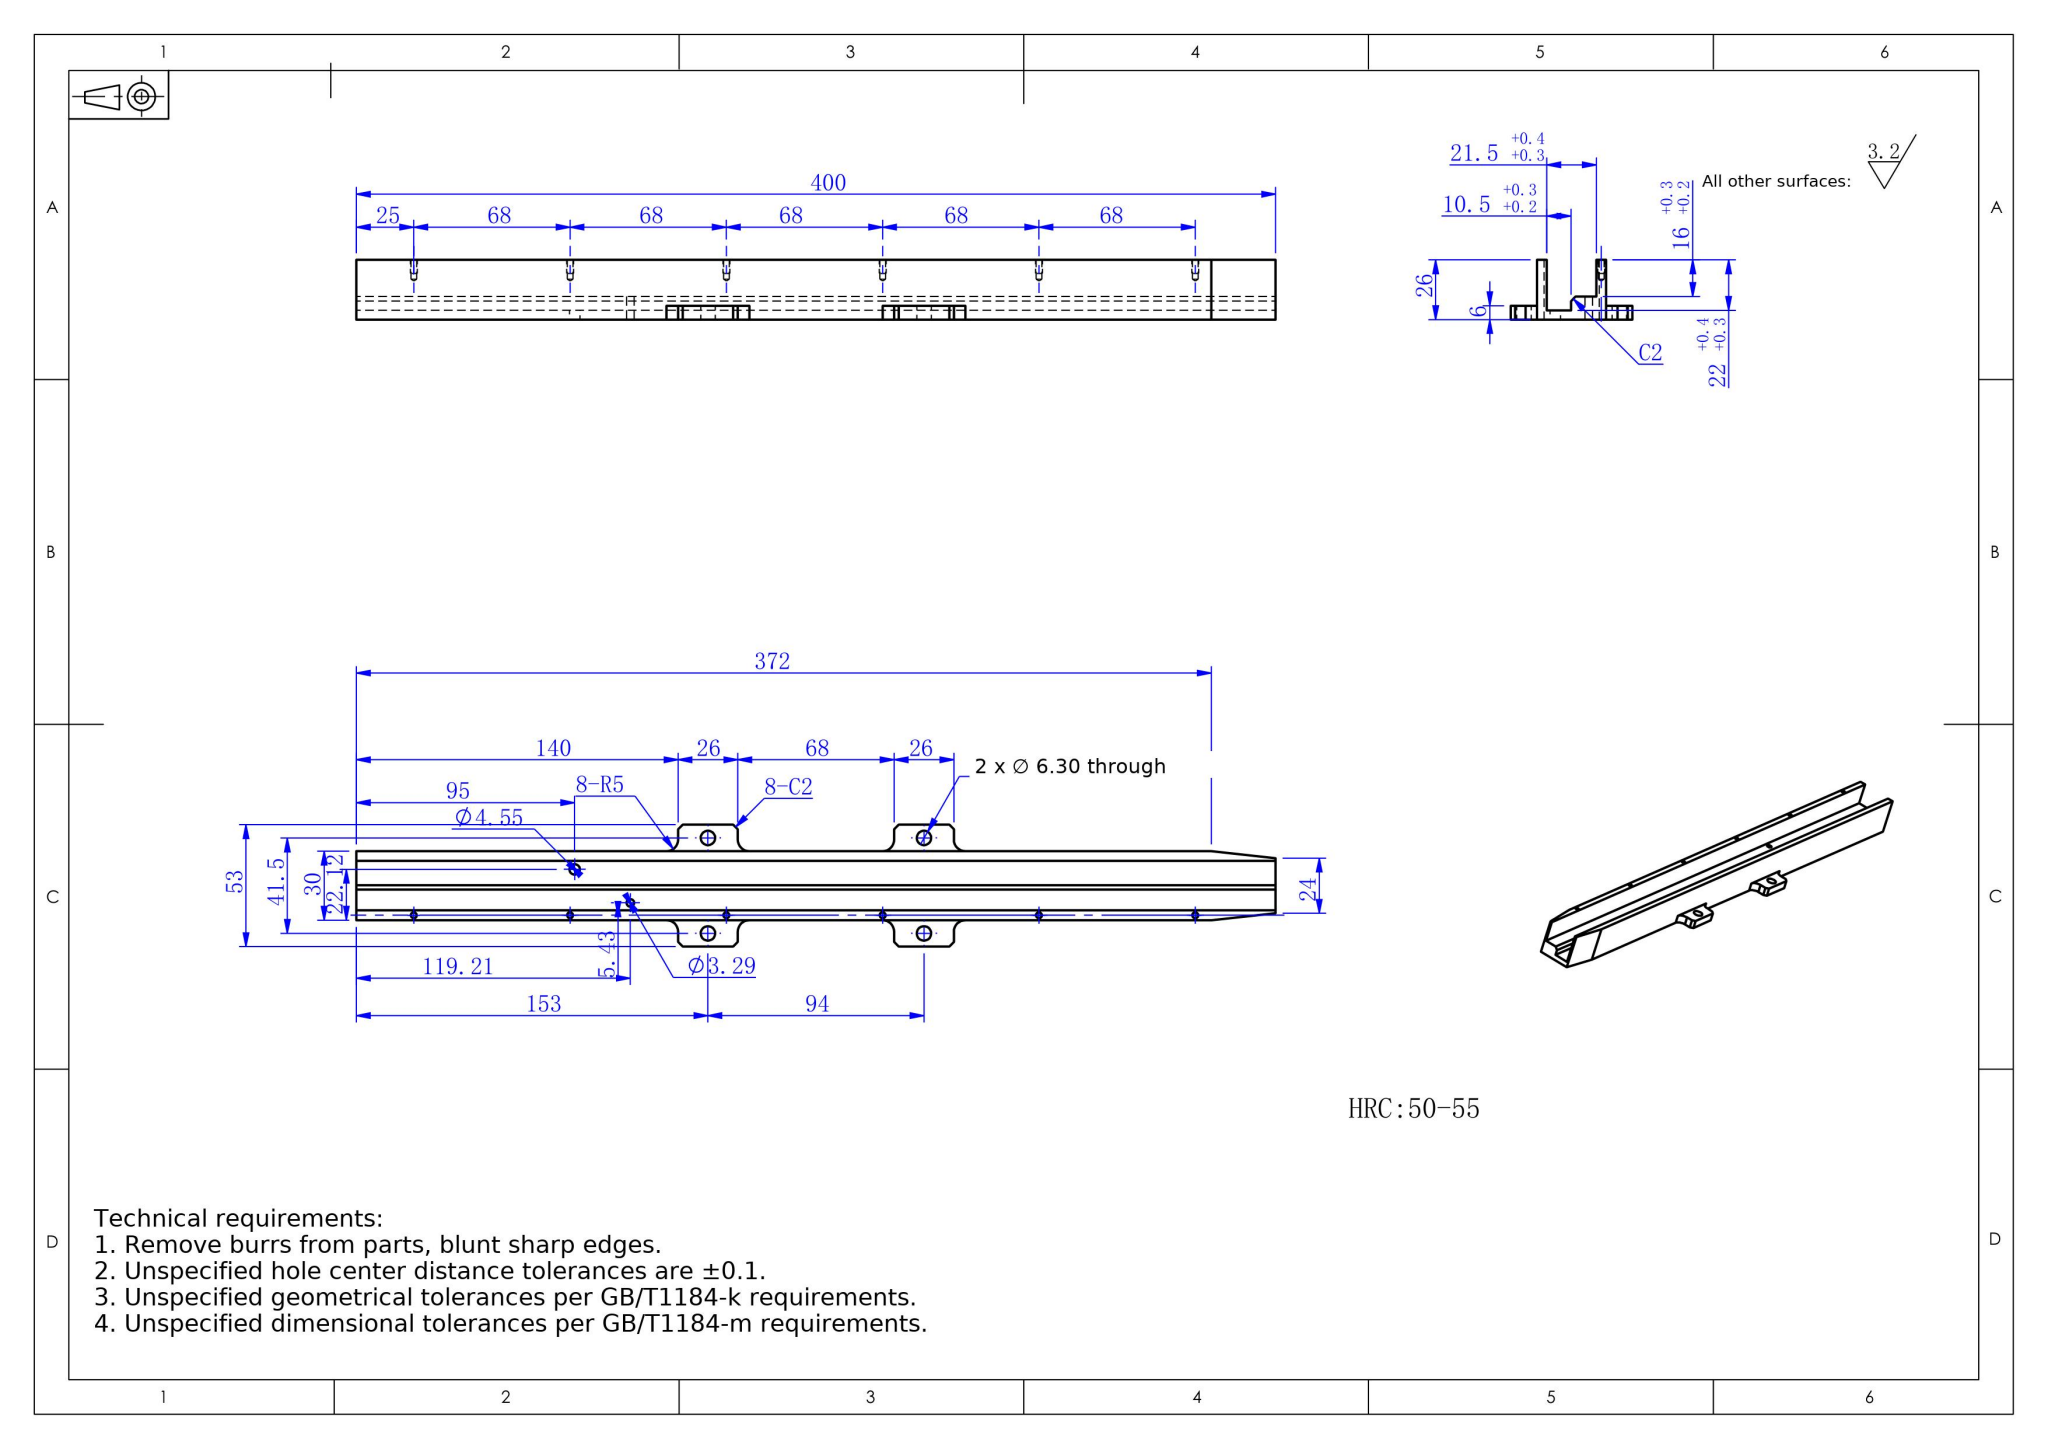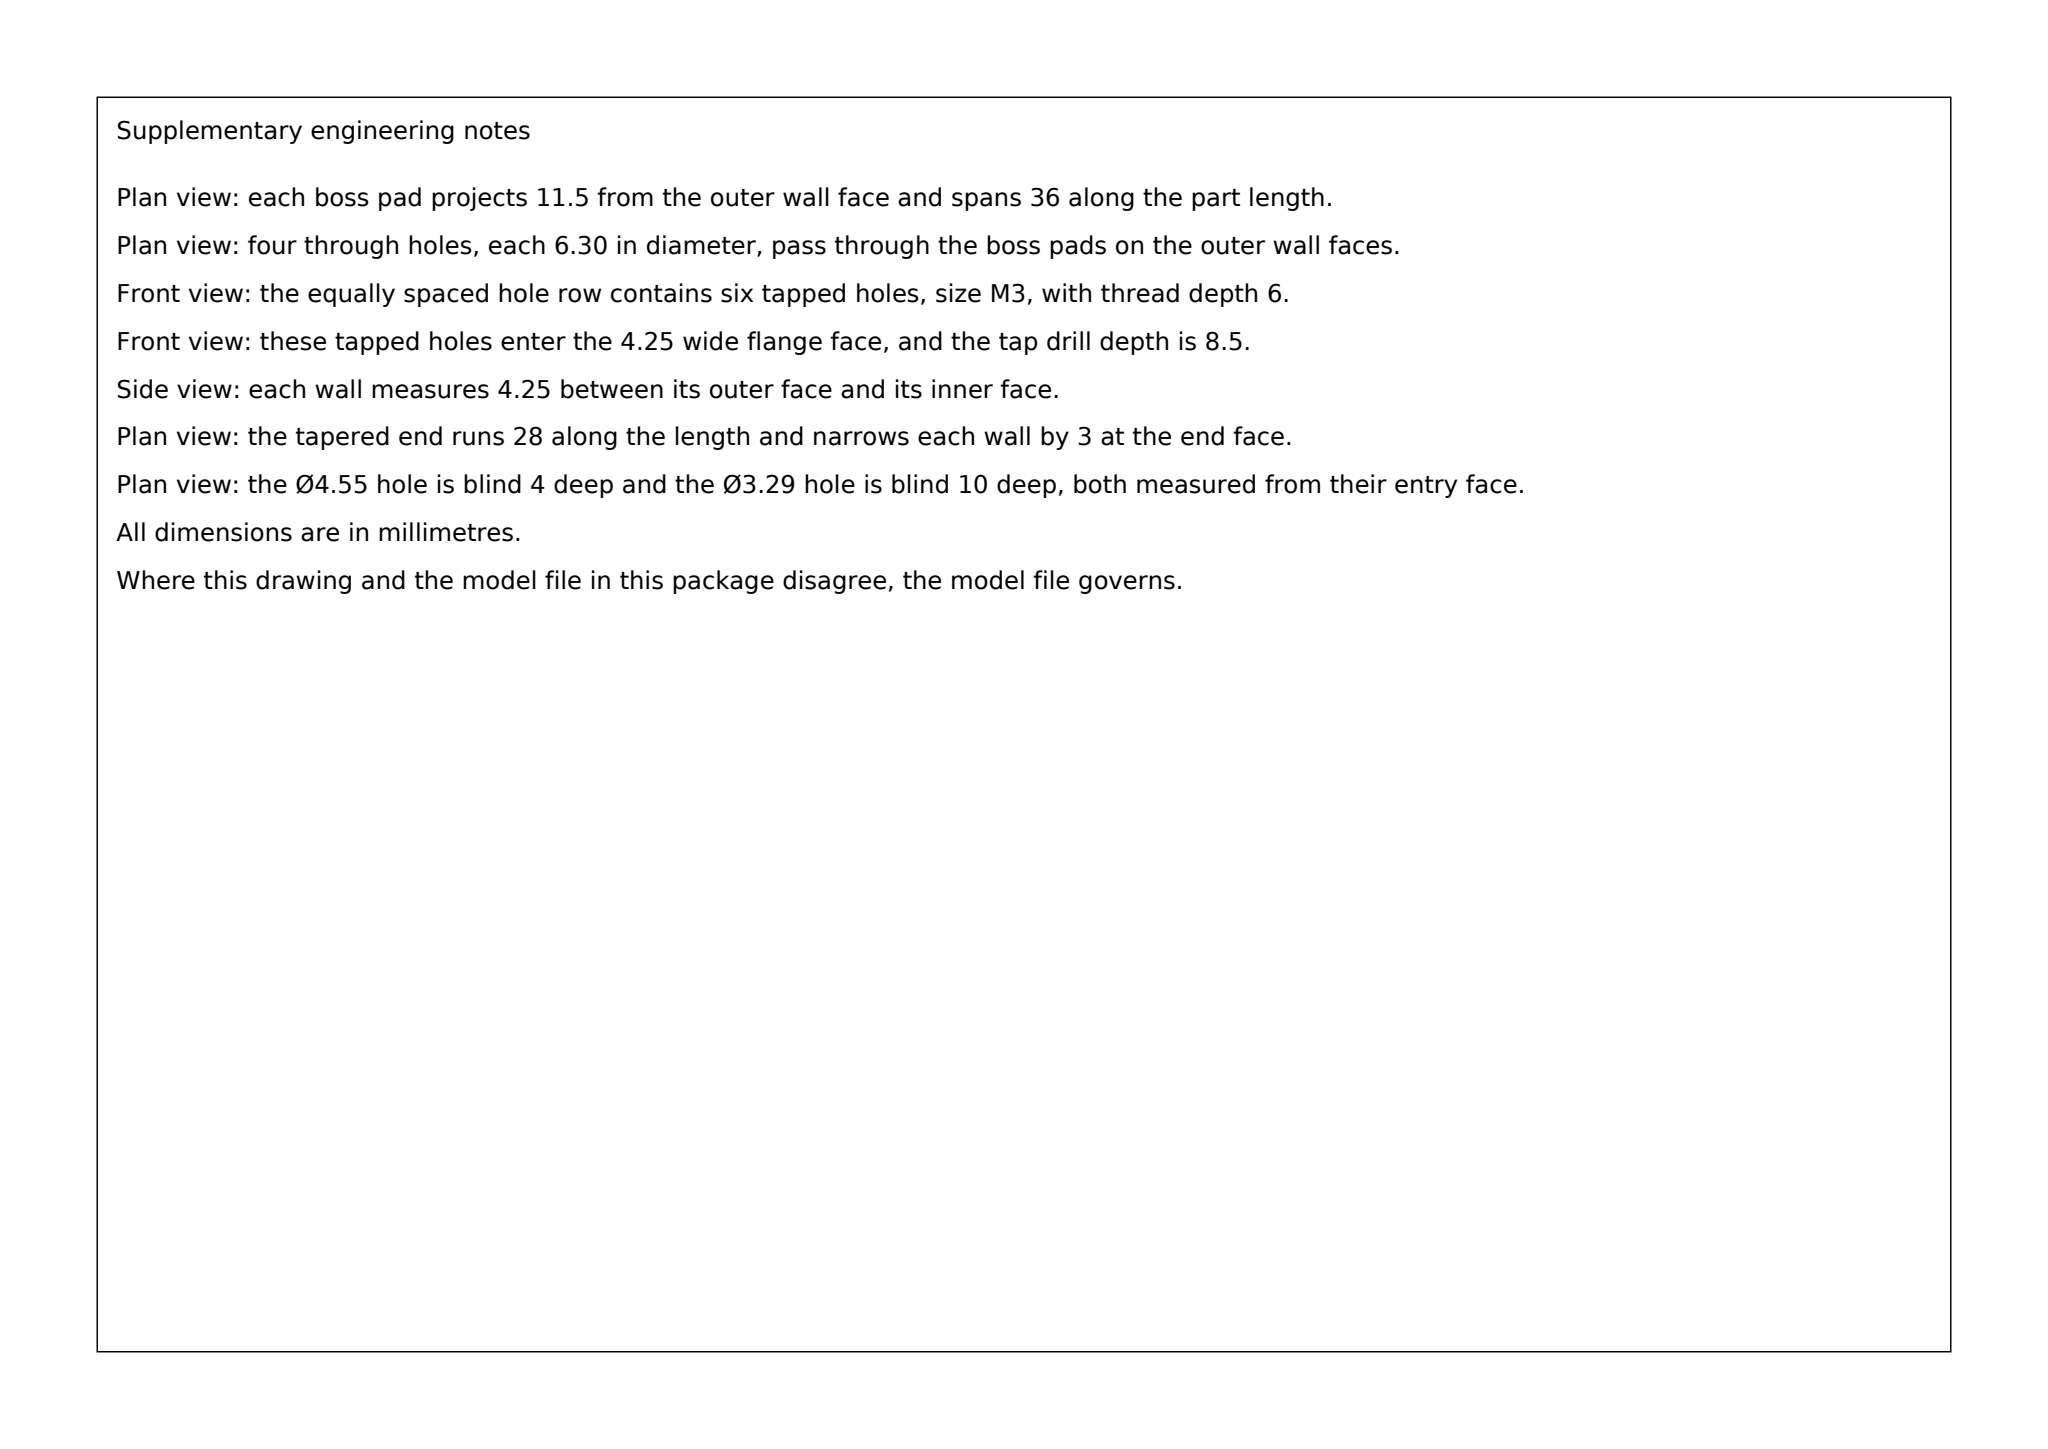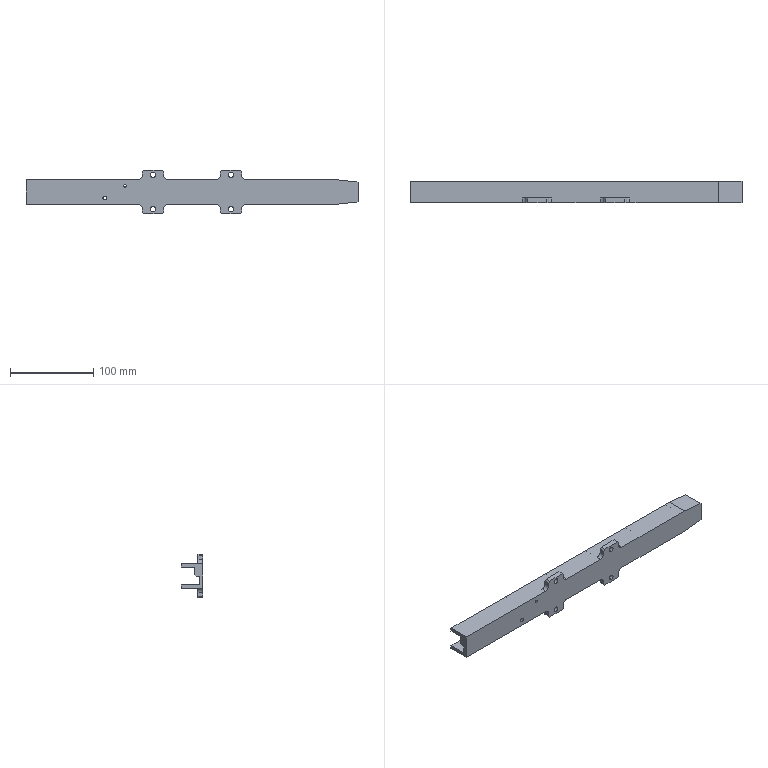Part | SolidWorks | mm | 1 solid | 83 faces | box 400 x 26 x 53 mm | volume 152398 mm3 | plane 39 | cylinder 32 | cone 12 | commonest cylinder face diameters 2.5 x12 6.3 x8 10 x8 4.55 x2 3.289 x2
Drawing notes:
12 x Ø2.5 DP 8.5, SPACED PER 25 & 68 DIMS, FRONT VIEW | from the solid: cylinders dia 2.5, axis y, len 8.5 at x=25,93,161,229,297,365 (count 2 ea)
Ø2.5 HOLES: 118° DRILL PT, FULL DIA DEPTH 8.5 | from the solid: cones[included_angle 118.0, ref_dia 2.5, qty 12]; cyl len 8.5
Ø2.5 HOLE ROW 39.38 FROM EDGE USED FOR 41.5 DIM, PLAN | from the solid: Ø2.5 cyl z-pos 39.38; z=0 bbox edge is origin of 53 and 41.5 dims
Ø3.29 HOLE 33.95 FROM EDGE USED FOR 41.5 DIM, PLAN | from the solid: Ø3.289 cyl at z=33.95; 39.38-33.95=5.43 matches chain dim
Ø4.55 DP 4 (BLIND) | from the solid: cylinder [4.55, y, x=95, z=19.38, length 4.0]
Ø3.29 DP 10 (BLIND) | from the solid: cylinder [3.289, y, x=119.21, z=33.95, length 10.0]
4 x Ø6.30 THRU 6 THK BASE ( DP 6) | from the solid: 4 cyl dia 6.3, len 6.0 at x=153/247, z=5.75/47.25; base y=0 to 6
SECT: 10.5 & 21.5 FROM FACE 15.75 OFF 53-WIDTH EDGE | from the solid: z planes 15.75, 26.25 (=15.75+10.5), 37.25 (=15.75+21.5)
SECT: RIB THK 11 (FACES Z26.25 & Z37.25); BASE THK 6 | from the solid: z planes 26.25 & 37.25 (diff 11); y planes 0 and 6
4 x Ø6.30: 5.75 FROM EA LONG EDGE, 41.5 APART, SYM ABT C/L | from the solid: Ø6.3 cyls at z=5.75 & 47.25 (x=153, 247); bbox width z=53, spacing 41.5
build123d program:
from build123d import *

# Parameters (mm, degrees)
SKETCH1_W                  = 400
SKETCH1_H                  = 26
BOSS_EXTRUDE1_DEPTH        = 30
SKETCH2_W                  = 21.5
SKETCH2_H                  = 22
CUT_EXTRUDE1_DEPTH         = 403.933
SKETCH3_W                  = 11
SKETCH3_H                  = 6
BOSS_EXTRUDE2_DEPTH        = 400
CHAMFER1_SIZE              = 2
CUT_EXTRUDE2_REACH         = 312.914
M3_TAPPED_HOLE1_D          = 2.5
M3_TAPPED_HOLE1_DEPTH      = 8.5
M3_TAPPED_HOLE1_TIP        = 0.7511
SKETCH7_W                  = 26
SKETCH7_H                  = 6
BOSS_EXTRUDE3_DEPTH        = 11.5
F_6_3_6_3_DIAMETER_HOLE1_D = 6.3
CHAMFER2_SIZE              = 2
FILLET1_R                  = 5
SKETCH10_R                 = 1.644
SKETCH10_R_2               = 2.275
CUT_EXTRUDE3_DEPTH         = 80


with BuildPart() as part:
    # Sketch1 → Boss-Extrude1 (new body)
    with BuildSketch(Plane.XY):
        with Locations((108.369, 25.147)):
            Rectangle(SKETCH1_W, SKETCH1_H)
    extrude(amount=BOSS_EXTRUDE1_DEPTH)

    # Sketch2 → Cut-Extrude1 (cut, through all)
    with BuildSketch(Plane(origin=(308.369, 0, 0), x_dir=(0, 0, -1), z_dir=(1, 0, 0))):
        with Locations((-15, 27.147)):
            Rectangle(SKETCH2_W, SKETCH2_H)
    extrude(amount=-CUT_EXTRUDE1_DEPTH, mode=Mode.SUBTRACT)

    # Sketch3 → Boss-Extrude2 (add)
    with BuildSketch(Plane(origin=(308.369, 0, 0), x_dir=(0, 0, -1), z_dir=(1, 0, 0))):
        with Locations((-20.25, 19.147)):
            Rectangle(SKETCH3_W, SKETCH3_H)
    extrude(amount=-BOSS_EXTRUDE2_DEPTH)

    # Chamfer1
    chamfer1_edges = [part.edges().sort_by_distance(p)[0] for p in [
        (108.369, 22.147, 14.75),
    ]]
    chamfer(chamfer1_edges, length=CHAMFER1_SIZE)

    # Sketch4 → Cut-Extrude2 (cut, up to next)
    with BuildSketch(Plane(origin=(0, 38.147, 0), x_dir=(1, 0, 0), z_dir=(0, 1, 0)), mode=Mode.PRIVATE) as cut_extrude2_sk1:
        Polygon((308.369, -3), (280.369, 0), (308.369, 0), align=None)
    cut_extrude2_tool1 = extrude(cut_extrude2_sk1.sketch, amount=-CUT_EXTRUDE2_REACH, mode=Mode.PRIVATE) & part.part
    # Sketch4 → Cut-Extrude2 (cut, up to next)
    with BuildSketch(Plane(origin=(0, 38.147, 0), x_dir=(1, 0, 0), z_dir=(0, 1, 0)), mode=Mode.PRIVATE) as cut_extrude2_sk2:
        Polygon((308.369, -27), (280.369, -30), (308.369, -30), align=None)
    cut_extrude2_tool2 = extrude(cut_extrude2_sk2.sketch, amount=-CUT_EXTRUDE2_REACH, mode=Mode.PRIVATE) & part.part
    add(cut_extrude2_tool1.solids().sort_by_distance((299.036, 38.147, 1))[0], mode=Mode.SUBTRACT)
    add(cut_extrude2_tool2.solids().sort_by_distance((299.036, 38.147, 29))[0], mode=Mode.SUBTRACT)

    # M3 Tapped Hole1
    with Locations(Plane(origin=(0, 38.147, 0), x_dir=(1, 0, 0), z_dir=(0, 1, 0))):
        with Locations((273.369, -27.875), (205.369, -27.875), (137.369, -27.875), (69.369, -27.875), (1.369, -27.875), (-66.631, -27.875)):
            Hole(M3_TAPPED_HOLE1_D / 2, depth=M3_TAPPED_HOLE1_DEPTH)
            with Locations((0, 0, -(M3_TAPPED_HOLE1_DEPTH + M3_TAPPED_HOLE1_TIP / 2))):  # 118° drill point
                Cone(0, M3_TAPPED_HOLE1_D / 2, M3_TAPPED_HOLE1_TIP, mode=Mode.SUBTRACT)

    # Sketch7 → Boss-Extrude3 (add)
    with BuildSketch(Plane(origin=(0, 0, 0), x_dir=(-1, 0, 0), z_dir=(0, 0, -1))):
        with Locations((-155.369, 15.147)):
            Rectangle(SKETCH7_W, SKETCH7_H)
        with Locations((-61.369, 15.147)):
            Rectangle(SKETCH7_W, SKETCH7_H)
    boss_extrude3 = extrude(amount=BOSS_EXTRUDE3_DEPTH)

    # 6.3 _6.3_ Diameter Hole1 (through all)
    with Locations(Plane(origin=(0, 18.147, 0), x_dir=(1, 0, 0), z_dir=(0, 1, 0))):
        with Locations((155.369, 5.75), (61.369, 5.75)):
            f_6_3_6_3_diameter_hole1 = Hole(F_6_3_6_3_DIAMETER_HOLE1_D / 2)

    # Mirror1: Boss-Extrude3, 6.3 _6.3_ Diameter Hole1 across plane
    add(boss_extrude3.mirror(Plane(origin=(0, 0, 15), x_dir=(1, 0, 0), z_dir=(0, 0, -1))))
    add(f_6_3_6_3_diameter_hole1.mirror(Plane(origin=(0, 0, 15), x_dir=(1, 0, 0), z_dir=(0, 0, -1))), mode=Mode.SUBTRACT)

    # Chamfer2
    chamfer2_edges = [part.edges().sort_by_distance(p)[0] for p in [
        (142.369, 15.147, -11.5),
        (168.369, 15.147, -11.5),
        (74.369, 15.147, -11.5),
        (48.369, 15.147, -11.5),
        (168.369, 15.147, 41.5),
        (142.369, 15.147, 41.5),
        (74.369, 15.147, 41.5),
        (48.369, 15.147, 41.5),
    ]]
    chamfer(chamfer2_edges, length=CHAMFER2_SIZE)

    # Fillet1
    fillet1_edges = [part.edges().sort_by_distance(p)[0] for p in [
        (142.369, 15.147, 30),
        (168.369, 15.147, 30),
        (74.369, 15.147, 30),
        (48.369, 15.147, 30),
        (168.369, 15.147, 0),
        (142.369, 15.147, 0),
        (74.369, 15.147, 0),
        (48.369, 15.147, 0),
    ]]
    fillet(fillet1_edges, radius=FILLET1_R)

    # Sketch10 → Cut-Extrude3 (cut)
    with BuildSketch(Plane(origin=(0, 22.147, 0), x_dir=(1, 0, 0), z_dir=(0, 1, 0))):
        with Locations(Location((27.579, -22.446, 0), (0, 0, 270))):
            Circle(SKETCH10_R)
        with Locations(Location((3.372, -7.881, 0), (0, 0, 270))):
            Circle(SKETCH10_R_2)
    extrude(amount=-CUT_EXTRUDE3_DEPTH, mode=Mode.SUBTRACT)


solid = part.part